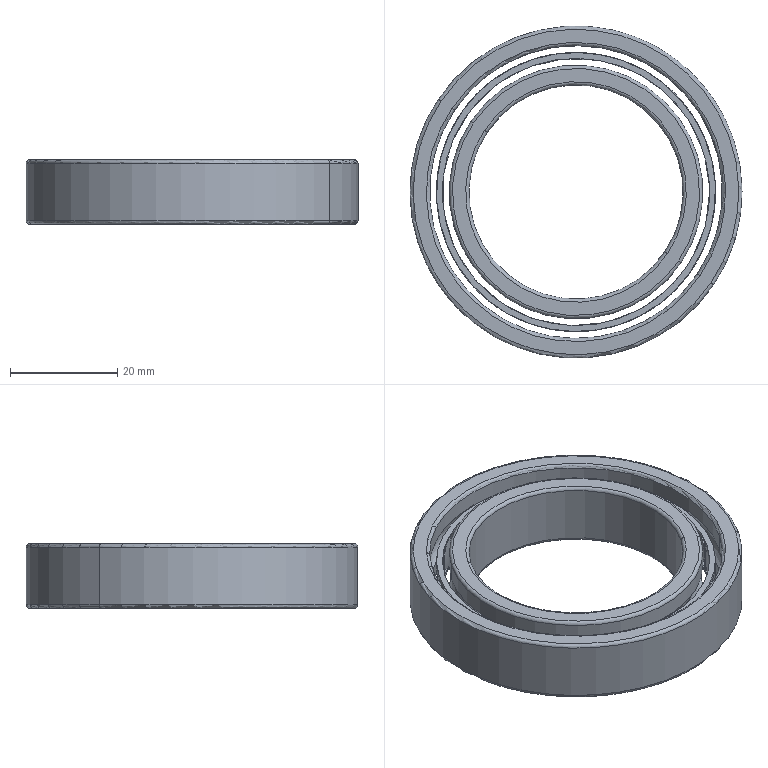Component | SolidWorks | MirrorDriveDevice-2_Mirrorgb_t276-2013[DeepGrooveBallBearing[60000]61908]-1 | 26 solids | 278 faces | volume 13744 mm3 | cylinder 112 | sphere 92 | plane 52 | torus 22 | commonest cylinder face diameters 6.15 x48 49.9 x26 52.1 x26 47.333 x4 54.667 x4 40 x2 62 x2